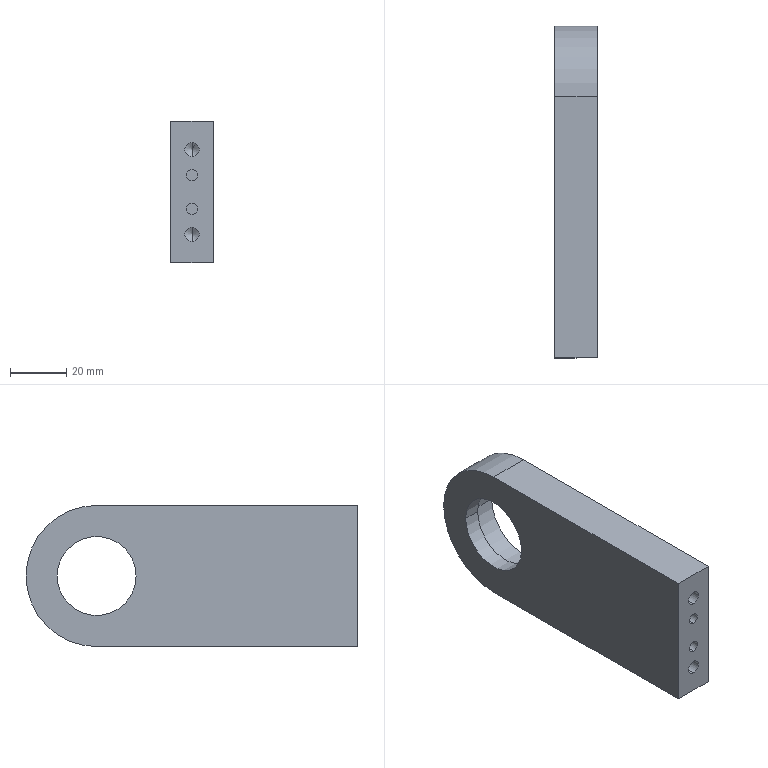Component | SolidWorks | 02-1 | 1 solid | 25 faces | box 15 x 117.6 x 50 mm | volume 72305 mm3 | cylinder 13 | plane 8 | cone 4 | commonest cylinder face diameters 4 x4 5 x4 32 x2 28 x2 50 x1
build123d program:
from build123d import *

# Parameters (mm, degrees)
SKETCH1_W             = 50
SKETCH1_H             = 117.6
EXTRUDE1_DEPTH        = 7.5
EXTRUDE3_DEPTH        = 66.631
SKETCH2_R             = 14
EXTRUDE2_DEPTH        = 66.631
SKETCH8_R             = 16
CUT_EXTRUDE1_DEPTH    = 9
M6_TAPPED_HOLE1_D     = 5
M6_TAPPED_HOLE1_DEPTH = 17
M6_TAPPED_HOLE1_TIP   = 1.502
SKETCH3_2_R           = 2
CUT_EXTRUDE1_2_DEPTH  = 10


with BuildPart() as part:
    # Sketch1 → Extrude1 (new, symmetric)
    with BuildSketch(Plane(origin=(0, 0, 0), x_dir=(1, 0, 0), z_dir=(0, 1, 0))):
        Rectangle(SKETCH1_W, SKETCH1_H)
    extrude(amount=EXTRUDE1_DEPTH, both=True)

    # Sketch3 → Extrude3 (cut, through all)
    with BuildSketch(Plane(origin=(0, 7.5, 0), x_dir=(1, 0, 0), z_dir=(0, 1, 0))):
        with BuildLine():
            ThreePointArc((0, 58.8), (17.678, 51.478), (25, 33.8))
            Line((25, 33.8), (25, 58.8))
            Line((25, 58.8), (0, 58.8))
        make_face()
        with BuildLine():
            ThreePointArc((-25, 33.8), (-17.678, 51.478), (0, 58.8))
            Line((0, 58.8), (-25, 58.8))
            Line((-25, 58.8), (-25, 33.8))
        make_face()
    extrude(amount=-EXTRUDE3_DEPTH, mode=Mode.SUBTRACT)

    # Sketch2 → Extrude2 (cut, through all)
    with BuildSketch(Plane(origin=(0, 7.5, 0), x_dir=(1, 0, 0), z_dir=(0, 1, 0))):
        with Locations(Location((0, 33.8, 0), (0, 0, 270))):
            Circle(SKETCH2_R)
    extrude(amount=-EXTRUDE2_DEPTH, mode=Mode.SUBTRACT)

    # Sketch8 → Cut-Extrude1 (cut)
    with BuildSketch(Plane.XZ.offset(7.5)):
        with Locations(Location((0, -33.8, 0), (0, 0, 270))):
            Circle(SKETCH8_R)
    extrude(amount=-CUT_EXTRUDE1_DEPTH, mode=Mode.SUBTRACT)

    # M6 Tapped Hole1
    with Locations(Plane.XY.offset(58.8)):
        with Locations((15, 0), (-15, 0)):
            Hole(M6_TAPPED_HOLE1_D / 2, depth=M6_TAPPED_HOLE1_DEPTH)
            with Locations((0, 0, -(M6_TAPPED_HOLE1_DEPTH + M6_TAPPED_HOLE1_TIP / 2))):  # 118° drill point
                Cone(0, M6_TAPPED_HOLE1_D / 2, M6_TAPPED_HOLE1_TIP, mode=Mode.SUBTRACT)

    # Sketch3_2 → Cut-Extrude1_2 (cut)
    with BuildSketch(Plane.XY.offset(58.8)):
        with Locations((6, 0)):
            Circle(SKETCH3_2_R)
        with Locations((-6, 0)):
            Circle(SKETCH3_2_R)
    extrude(amount=-CUT_EXTRUDE1_2_DEPTH, mode=Mode.SUBTRACT)


solid = part.part

# Placed as in the assembly
solid = solid.moved(Location((-87, -66.3, 30), (90, 0, 90)))
STEP:
#1=COLOUR_RGB('',0.7922,0.8196,0.9333);
#2=FILL_AREA_STYLE_COLOUR('',#1);
#3=FILL_AREA_STYLE('',(#2));
#4=SURFACE_STYLE_FILL_AREA(#3);
#5=SURFACE_SIDE_STYLE('',(#4));
#6=SURFACE_STYLE_USAGE(.BOTH.,#5);
#7=PRESENTATION_STYLE_ASSIGNMENT((#6));
#8=CARTESIAN_POINT('',(-3.425,-4.531,0.8661));
#9=VERTEX_POINT('',#8);
#10=CARTESIAN_POINT('',(-3.425,-4.531,1.024));
#11=VERTEX_POINT('',#10);
#12=CARTESIAN_POINT('',(-3.425,-4.531,0.9449));
#13=DIRECTION('',(0.,-1.,-0.));
#14=DIRECTION('',(0.,0.,1.));
#15=AXIS2_PLACEMENT_3D('',#12,#13,#14);
#16=CIRCLE('',#15,0.07874);
#17=EDGE_CURVE('',#9,#11,#16,.T.);
#18=ORIENTED_EDGE('',*,*,#17,.F.);
#19=CARTESIAN_POINT('',(-3.425,-4.925,0.8661));
#20=VERTEX_POINT('',#19);
#21=CARTESIAN_POINT('',(-3.425,-4.531,0.8661));
#22=DIRECTION('',(0.,-1.,-0.));
#23=VECTOR('',#22,39.37);
#24=LINE('',#21,#23);
#25=EDGE_CURVE('',#9,#20,#24,.T.);
#26=ORIENTED_EDGE('',*,*,#25,.T.);
#27=CARTESIAN_POINT('',(-3.425,-4.925,1.024));
#28=VERTEX_POINT('',#27);
#29=CARTESIAN_POINT('',(-3.425,-4.925,0.9449));
#30=DIRECTION('',(0.,-1.,-0.));
#31=DIRECTION('',(0.,0.,1.));
#32=AXIS2_PLACEMENT_3D('',#29,#30,#31);
#33=CIRCLE('',#32,0.07874);
#34=EDGE_CURVE('',#20,#28,#33,.T.);
#35=ORIENTED_EDGE('',*,*,#34,.T.);
#36=CARTESIAN_POINT('',(-3.425,-4.531,1.024));
#37=DIRECTION('',(0.,-1.,-0.));
#38=VECTOR('',#37,39.37);
#39=LINE('',#36,#38);
#40=EDGE_CURVE('',#11,#28,#39,.T.);
#41=ORIENTED_EDGE('',*,*,#40,.F.);
#42=EDGE_LOOP('',(#18,#26,#35,#41));
#43=FACE_OUTER_BOUND('',#42,.T.);
#44=CARTESIAN_POINT('',(-3.425,-4.531,0.9449));
#45=DIRECTION('',(0.,-1.,-0.));
#46=DIRECTION('',(0.,0.,1.));
#47=AXIS2_PLACEMENT_3D('',#44,#45,#46);
#48=CYLINDRICAL_SURFACE('',#47,0.07874);
#49=ADVANCED_FACE('',(#43),#48,.F.);
#50=CARTESIAN_POINT('',(-3.425,-4.531,1.339));
#51=VERTEX_POINT('',#50);
#52=CARTESIAN_POINT('',(-3.425,-4.531,1.496));
#53=VERTEX_POINT('',#52);
#54=CARTESIAN_POINT('',(-3.425,-4.531,1.417));
#55=DIRECTION('',(0.,-1.,-0.));
#56=DIRECTION('',(0.,0.,1.));
#57=AXIS2_PLACEMENT_3D('',#54,#55,#56);
#58=CIRCLE('',#57,0.07874);
#59=EDGE_CURVE('',#51,#53,#58,.T.);
#60=ORIENTED_EDGE('',*,*,#59,.F.);
#61=CARTESIAN_POINT('',(-3.425,-4.925,1.339));
#62=VERTEX_POINT('',#61);
#63=CARTESIAN_POINT('',(-3.425,-4.531,1.339));
#64=DIRECTION('',(0.,-1.,-0.));
#65=VECTOR('',#64,39.37);
#66=LINE('',#63,#65);
#67=EDGE_CURVE('',#51,#62,#66,.T.);
#68=ORIENTED_EDGE('',*,*,#67,.T.);
#69=CARTESIAN_POINT('',(-3.425,-4.925,1.496));
#70=VERTEX_POINT('',#69);
#71=CARTESIAN_POINT('',(-3.425,-4.925,1.417));
#72=DIRECTION('',(0.,-1.,-0.));
#73=DIRECTION('',(0.,0.,1.));
#74=AXIS2_PLACEMENT_3D('',#71,#72,#73);
#75=CIRCLE('',#74,0.07874);
#76=EDGE_CURVE('',#62,#70,#75,.T.);
#77=ORIENTED_EDGE('',*,*,#76,.T.);
#78=CARTESIAN_POINT('',(-3.425,-4.531,1.496));
#79=DIRECTION('',(0.,-1.,-0.));
#80=VECTOR('',#79,39.37);
#81=LINE('',#78,#80);
#82=EDGE_CURVE('',#53,#70,#81,.T.);
#83=ORIENTED_EDGE('',*,*,#82,.F.);
#84=EDGE_LOOP('',(#60,#68,#77,#83));
#85=FACE_OUTER_BOUND('',#84,.T.);
#86=CARTESIAN_POINT('',(-3.425,-4.531,1.417));
#87=DIRECTION('',(0.,-1.,-0.));
#88=DIRECTION('',(0.,0.,1.));
#89=AXIS2_PLACEMENT_3D('',#86,#87,#88);
#90=CYLINDRICAL_SURFACE('',#89,0.07874);
#91=ADVANCED_FACE('',(#85),#90,.F.);
#92=CARTESIAN_POINT('',(-3.425,-4.256,1.673));
#93=VERTEX_POINT('',#92);
#94=CARTESIAN_POINT('',(-3.425,-4.256,1.87));
#95=VERTEX_POINT('',#94);
#96=CARTESIAN_POINT('',(-3.425,-4.256,1.772));
#97=DIRECTION('',(0.,-1.,-0.));
#98=DIRECTION('',(0.,0.,1.));
#99=AXIS2_PLACEMENT_3D('',#96,#97,#98);
#100=CIRCLE('',#99,0.09843);
#101=EDGE_CURVE('',#93,#95,#100,.T.);
#102=ORIENTED_EDGE('',*,*,#101,.F.);
#103=CARTESIAN_POINT('',(-3.425,-4.925,1.673));
#104=VERTEX_POINT('',#103);
#105=CARTESIAN_POINT('',(-3.425,-4.925,1.673));
#106=DIRECTION('',(0.,-1.,-0.));
#107=VECTOR('',#106,39.37);
#108=LINE('',#105,#107);
#109=EDGE_CURVE('',#93,#104,#108,.T.);
#110=ORIENTED_EDGE('',*,*,#109,.T.);
#111=CARTESIAN_POINT('',(-3.425,-4.925,1.87));
#112=VERTEX_POINT('',#111);
#113=CARTESIAN_POINT('',(-3.425,-4.925,1.772));
#114=DIRECTION('',(0.,-1.,-0.));
#115=DIRECTION('',(0.,0.,1.));
#116=AXIS2_PLACEMENT_3D('',#113,#114,#115);
#117=CIRCLE('',#116,0.09843);
#118=EDGE_CURVE('',#104,#112,#117,.T.);
#119=ORIENTED_EDGE('',*,*,#118,.T.);
#120=CARTESIAN_POINT('',(-3.425,-4.925,1.87));
#121=DIRECTION('',(0.,-1.,-0.));
#122=VECTOR('',#121,39.37);
#123=LINE('',#120,#122);
#124=EDGE_CURVE('',#95,#112,#123,.T.);
#125=ORIENTED_EDGE('',*,*,#124,.F.);
#126=EDGE_LOOP('',(#102,#110,#119,#125));
#127=FACE_OUTER_BOUND('',#126,.T.);
#128=CARTESIAN_POINT('',(-3.425,-4.925,1.772));
#129=DIRECTION('',(0.,-1.,-0.));
#130=DIRECTION('',(0.,0.,1.));
#131=AXIS2_PLACEMENT_3D('',#128,#129,#130);
#132=CYLINDRICAL_SURFACE('',#131,0.09843);
#133=ADVANCED_FACE('',(#127),#132,.F.);
#134=CARTESIAN_POINT('',(-3.425,-4.197,1.772));
#135=VERTEX_POINT('',#134);
#136=CARTESIAN_POINT('',(-3.425,-4.256,1.87));
#137=DIRECTION('',(0.,-0.515,0.8572));
#138=VECTOR('',#137,39.37);
#139=LINE('',#136,#138);
#140=EDGE_CURVE('',#135,#95,#139,.T.);
#141=ORIENTED_EDGE('',*,*,#140,.F.);
#142=CARTESIAN_POINT('',(-3.425,-4.256,1.673));
#143=DIRECTION('',(-0.,-0.515,-0.8572));
#144=VECTOR('',#143,39.37);
#145=LINE('',#142,#144);
#146=EDGE_CURVE('',#135,#93,#145,.T.);
#147=ORIENTED_EDGE('',*,*,#146,.T.);
#148=ORIENTED_EDGE('',*,*,#101,.T.);
#149=EDGE_LOOP('',(#141,#147,#148));
#150=FACE_OUTER_BOUND('',#149,.T.);
#151=CARTESIAN_POINT('',(-3.425,-4.256,1.772));
#152=DIRECTION('',(0.,-1.,-0.));
#153=DIRECTION('',(0.,0.,1.));
#154=AXIS2_PLACEMENT_3D('',#151,#152,#153);
#155=CONICAL_SURFACE('',#154,0.09843,1.03);
#156=ADVANCED_FACE('',(#150),#155,.F.);
#157=CARTESIAN_POINT('',(-3.425,-4.256,0.4921));
#158=VERTEX_POINT('',#157);
#159=CARTESIAN_POINT('',(-3.425,-4.256,0.689));
#160=VERTEX_POINT('',#159);
#161=CARTESIAN_POINT('',(-3.425,-4.256,0.5906));
#162=DIRECTION('',(0.,-1.,-0.));
#163=DIRECTION('',(0.,0.,1.));
#164=AXIS2_PLACEMENT_3D('',#161,#162,#163);
#165=CIRCLE('',#164,0.09843);
#166=EDGE_CURVE('',#158,#160,#165,.T.);
#167=ORIENTED_EDGE('',*,*,#166,.F.);
#168=CARTESIAN_POINT('',(-3.425,-4.925,0.4921));
#169=VERTEX_POINT('',#168);
#170=CARTESIAN_POINT('',(-3.425,-4.925,0.4921));
#171=DIRECTION('',(0.,-1.,-0.));
#172=VECTOR('',#171,39.37);
#173=LINE('',#170,#172);
#174=EDGE_CURVE('',#158,#169,#173,.T.);
#175=ORIENTED_EDGE('',*,*,#174,.T.);
#176=CARTESIAN_POINT('',(-3.425,-4.925,0.689));
#177=VERTEX_POINT('',#176);
#178=CARTESIAN_POINT('',(-3.425,-4.925,0.5906));
#179=DIRECTION('',(0.,-1.,-0.));
#180=DIRECTION('',(0.,0.,1.));
#181=AXIS2_PLACEMENT_3D('',#178,#179,#180);
#182=CIRCLE('',#181,0.09843);
#183=EDGE_CURVE('',#169,#177,#182,.T.);
#184=ORIENTED_EDGE('',*,*,#183,.T.);
#185=CARTESIAN_POINT('',(-3.425,-4.925,0.689));
#186=DIRECTION('',(0.,-1.,-0.));
#187=VECTOR('',#186,39.37);
#188=LINE('',#185,#187);
#189=EDGE_CURVE('',#160,#177,#188,.T.);
#190=ORIENTED_EDGE('',*,*,#189,.F.);
#191=EDGE_LOOP('',(#167,#175,#184,#190));
#192=FACE_OUTER_BOUND('',#191,.T.);
#193=CARTESIAN_POINT('',(-3.425,-4.925,0.5906));
#194=DIRECTION('',(0.,-1.,-0.));
#195=DIRECTION('',(0.,0.,1.));
#196=AXIS2_PLACEMENT_3D('',#193,#194,#195);
#197=CYLINDRICAL_SURFACE('',#196,0.09843);
#198=ADVANCED_FACE('',(#192),#197,.F.);
#199=CARTESIAN_POINT('',(-3.425,-4.197,0.5906));
#200=VERTEX_POINT('',#199);
#201=CARTESIAN_POINT('',(-3.425,-4.256,0.689));
#202=DIRECTION('',(0.,-0.515,0.8572));
#203=VECTOR('',#202,39.37);
#204=LINE('',#201,#203);
#205=EDGE_CURVE('',#200,#160,#204,.T.);
#206=ORIENTED_EDGE('',*,*,#205,.F.);
#207=CARTESIAN_POINT('',(-3.425,-4.256,0.4921));
#208=DIRECTION('',(-0.,-0.515,-0.8572));
#209=VECTOR('',#208,39.37);
#210=LINE('',#207,#209);
#211=EDGE_CURVE('',#200,#158,#210,.T.);
#212=ORIENTED_EDGE('',*,*,#211,.T.);
#213=ORIENTED_EDGE('',*,*,#166,.T.);
#214=EDGE_LOOP('',(#206,#212,#213));
#215=FACE_OUTER_BOUND('',#214,.T.);
#216=CARTESIAN_POINT('',(-3.425,-4.256,0.5906));
#217=DIRECTION('',(0.,-1.,-0.));
#218=DIRECTION('',(0.,0.,1.));
#219=AXIS2_PLACEMENT_3D('',#216,#217,#218);
#220=CONICAL_SURFACE('',#219,0.09843,1.03);
#221=ADVANCED_FACE('',(#215),#220,.F.);
#222=CARTESIAN_POINT('',(-3.484,-1.909,1.181));
#223=VERTEX_POINT('',#222);
#224=CARTESIAN_POINT('',(-3.484,-0.6496,1.181));
#225=VERTEX_POINT('',#224);
#226=CARTESIAN_POINT('',(-3.484,-1.28,1.181));
#227=DIRECTION('',(1.,0.,-0.));
#228=DIRECTION('',(0.,1.,0.));
#229=AXIS2_PLACEMENT_3D('',#226,#227,#228);
#230=CIRCLE('',#229,0.6299);
#231=EDGE_CURVE('',#223,#225,#230,.T.);
#232=ORIENTED_EDGE('',*,*,#231,.F.);
#233=CARTESIAN_POINT('',(-3.13,-1.909,1.181));
#234=VERTEX_POINT('',#233);
#235=CARTESIAN_POINT('',(-3.484,-1.909,1.181));
#236=DIRECTION('',(1.,0.,-0.));
#237=VECTOR('',#236,39.37);
#238=LINE('',#235,#237);
#239=EDGE_CURVE('',#223,#234,#238,.T.);
#240=ORIENTED_EDGE('',*,*,#239,.T.);
#241=CARTESIAN_POINT('',(-3.13,-0.6496,1.181));
#242=VERTEX_POINT('',#241);
#243=CARTESIAN_POINT('',(-3.13,-1.28,1.181));
#244=DIRECTION('',(1.,0.,-0.));
#245=DIRECTION('',(0.,1.,0.));
#246=AXIS2_PLACEMENT_3D('',#243,#244,#245);
#247=CIRCLE('',#246,0.6299);
#248=EDGE_CURVE('',#234,#242,#247,.T.);
#249=ORIENTED_EDGE('',*,*,#248,.T.);
#250=CARTESIAN_POINT('',(-3.484,-0.6496,1.181));
#251=DIRECTION('',(1.,0.,-0.));
#252=VECTOR('',#251,39.37);
#253=LINE('',#250,#252);
#254=EDGE_CURVE('',#225,#242,#253,.T.);
#255=ORIENTED_EDGE('',*,*,#254,.F.);
#256=EDGE_LOOP('',(#232,#240,#249,#255));
#257=FACE_OUTER_BOUND('',#256,.T.);
#258=CARTESIAN_POINT('',(-3.484,-1.28,1.181));
#259=DIRECTION('',(1.,0.,-0.));
#260=DIRECTION('',(0.,1.,0.));
#261=AXIS2_PLACEMENT_3D('',#258,#259,#260);
#262=CYLINDRICAL_SURFACE('',#261,0.6299);
#263=ADVANCED_FACE('',(#257),#262,.F.);
#264=CARTESIAN_POINT('',(-3.484,-0.7283,1.181));
#265=VERTEX_POINT('',#264);
#266=CARTESIAN_POINT('',(-3.484,-1.831,1.181));
#267=VERTEX_POINT('',#266);
#268=CARTESIAN_POINT('',(-3.484,-1.28,1.181));
#269=DIRECTION('',(-1.,-0.,0.));
#270=DIRECTION('',(0.,1.,0.));
#271=AXIS2_PLACEMENT_3D('',#268,#269,#270);
#272=CIRCLE('',#271,0.5512);
#273=EDGE_CURVE('',#265,#267,#272,.T.);
#274=ORIENTED_EDGE('',*,*,#273,.F.);
#275=CARTESIAN_POINT('',(-3.72,-0.7283,1.181));
#276=VERTEX_POINT('',#275);
#277=CARTESIAN_POINT('',(-3.13,-0.7283,1.181));
#278=DIRECTION('',(-1.,-0.,0.));
#279=VECTOR('',#278,39.37);
#280=LINE('',#277,#279);
#281=EDGE_CURVE('',#265,#276,#280,.T.);
#282=ORIENTED_EDGE('',*,*,#281,.T.);
#283=CARTESIAN_POINT('',(-3.72,-1.831,1.181));
#284=VERTEX_POINT('',#283);
#285=CARTESIAN_POINT('',(-3.72,-1.28,1.181));
#286=DIRECTION('',(-1.,-0.,0.));
#287=DIRECTION('',(0.,-1.,0.));
#288=AXIS2_PLACEMENT_3D('',#285,#286,#287);
#289=CIRCLE('',#288,0.5512);
#290=EDGE_CURVE('',#276,#284,#289,.T.);
#291=ORIENTED_EDGE('',*,*,#290,.T.);
#292=CARTESIAN_POINT('',(-3.13,-1.831,1.181));
#293=DIRECTION('',(-1.,-0.,0.));
#294=VECTOR('',#293,39.37);
#295=LINE('',#292,#294);
#296=EDGE_CURVE('',#267,#284,#295,.T.);
#297=ORIENTED_EDGE('',*,*,#296,.F.);
#298=EDGE_LOOP('',(#274,#282,#291,#297));
#299=FACE_OUTER_BOUND('',#298,.T.);
#300=CARTESIAN_POINT('',(-3.13,-1.28,1.181));
#301=DIRECTION('',(-1.,-0.,0.));
#302=DIRECTION('',(0.,-1.,0.));
#303=AXIS2_PLACEMENT_3D('',#300,#301,#302);
#304=CYLINDRICAL_SURFACE('',#303,0.5512);
#305=ADVANCED_FACE('',(#299),#304,.F.);
#306=ORIENTED_EDGE('',*,*,#281,.F.);
#307=CARTESIAN_POINT('',(-3.484,-1.28,1.181));
#308=DIRECTION('',(-1.,-0.,0.));
#309=DIRECTION('',(0.,1.,0.));
#310=AXIS2_PLACEMENT_3D('',#307,#308,#309);
#311=CIRCLE('',#310,0.5512);
#312=EDGE_CURVE('',#267,#265,#311,.T.);
#313=ORIENTED_EDGE('',*,*,#312,.F.);
#314=ORIENTED_EDGE('',*,*,#296,.T.);
#315=CARTESIAN_POINT('',(-3.72,-1.28,1.181));
#316=DIRECTION('',(-1.,-0.,0.));
#317=DIRECTION('',(0.,-1.,0.));
#318=AXIS2_PLACEMENT_3D('',#315,#316,#317);
#319=CIRCLE('',#318,0.5512);
#320=EDGE_CURVE('',#284,#276,#319,.T.);
#321=ORIENTED_EDGE('',*,*,#320,.T.);
#322=EDGE_LOOP('',(#306,#313,#314,#321));
#323=FACE_OUTER_BOUND('',#322,.T.);
#324=CARTESIAN_POINT('',(-3.13,-1.28,1.181));
#325=DIRECTION('',(-1.,-0.,0.));
#326=DIRECTION('',(0.,-1.,0.));
#327=AXIS2_PLACEMENT_3D('',#324,#325,#326);
#328=CYLINDRICAL_SURFACE('',#327,0.5512);
#329=ADVANCED_FACE('',(#323),#328,.F.);
#330=ORIENTED_EDGE('',*,*,#320,.F.);
#331=ORIENTED_EDGE('',*,*,#290,.F.);
#332=EDGE_LOOP('',(#330,#331));
#333=FACE_BOUND('',#332,.T.);
#334=CARTESIAN_POINT('',(-3.72,-4.925,2.165));
#335=VERTEX_POINT('',#334);
#336=CARTESIAN_POINT('',(-3.72,-1.28,2.165));
#337=VERTEX_POINT('',#336);
#338=CARTESIAN_POINT('',(-3.72,-0.2953,2.165));
#339=DIRECTION('',(-0.,1.,0.));
#340=VECTOR('',#339,39.37);
#341=LINE('',#338,#340);
#342=EDGE_CURVE('',#335,#337,#341,.T.);
#343=ORIENTED_EDGE('',*,*,#342,.T.);
#344=CARTESIAN_POINT('',(-3.72,-1.28,0.1969));
#345=VERTEX_POINT('',#344);
#346=CARTESIAN_POINT('',(-3.72,-1.28,1.181));
#347=DIRECTION('',(-1.,-0.,0.));
#348=DIRECTION('',(0.,-1.,-0.));
#349=AXIS2_PLACEMENT_3D('',#346,#347,#348);
#350=CIRCLE('',#349,0.9843);
#351=EDGE_CURVE('',#337,#345,#350,.T.);
#352=ORIENTED_EDGE('',*,*,#351,.T.);
#353=CARTESIAN_POINT('',(-3.72,-4.925,0.1969));
#354=VERTEX_POINT('',#353);
#355=CARTESIAN_POINT('',(-3.72,-0.2953,0.1969));
#356=DIRECTION('',(0.,-1.,-0.));
#357=VECTOR('',#356,39.37);
#358=LINE('',#355,#357);
#359=EDGE_CURVE('',#345,#354,#358,.T.);
#360=ORIENTED_EDGE('',*,*,#359,.T.);
#361=CARTESIAN_POINT('',(-3.72,-4.925,2.165));
#362=DIRECTION('',(0.,-0.,1.));
#363=VECTOR('',#362,39.37);
#364=LINE('',#361,#363);
#365=EDGE_CURVE('',#354,#335,#364,.T.);
#366=ORIENTED_EDGE('',*,*,#365,.T.);
#367=EDGE_LOOP('',(#343,#352,#360,#366));
#368=FACE_OUTER_BOUND('',#367,.T.);
#369=CARTESIAN_POINT('',(-3.72,-2.61,1.181));
#370=DIRECTION('',(1.,0.,-0.));
#371=DIRECTION('',(-0.,1.,0.));
#372=AXIS2_PLACEMENT_3D('',#369,#370,#371);
#373=PLANE('',#372);
#374=ADVANCED_FACE('',(#333,#368),#373,.F.);
#375=CARTESIAN_POINT('',(-3.13,-1.28,1.181));
#376=DIRECTION('',(1.,0.,-0.));
#377=DIRECTION('',(0.,1.,0.));
#378=AXIS2_PLACEMENT_3D('',#375,#376,#377);
#379=CIRCLE('',#378,0.6299);
#380=EDGE_CURVE('',#242,#234,#379,.T.);
#381=ORIENTED_EDGE('',*,*,#380,.F.);
#382=ORIENTED_EDGE('',*,*,#248,.F.);
#383=EDGE_LOOP('',(#381,#382));
#384=FACE_BOUND('',#383,.T.);
#385=CARTESIAN_POINT('',(-3.13,-1.28,2.165));
#386=VERTEX_POINT('',#385);
#387=CARTESIAN_POINT('',(-3.13,-1.28,0.1969));
#388=VERTEX_POINT('',#387);
#389=CARTESIAN_POINT('',(-3.13,-1.28,1.181));
#390=DIRECTION('',(-1.,-0.,0.));
#391=DIRECTION('',(0.,-1.,-0.));
#392=AXIS2_PLACEMENT_3D('',#389,#390,#391);
#393=CIRCLE('',#392,0.9843);
#394=EDGE_CURVE('',#386,#388,#393,.T.);
#395=ORIENTED_EDGE('',*,*,#394,.F.);
#396=CARTESIAN_POINT('',(-3.13,-4.925,2.165));
#397=VERTEX_POINT('',#396);
#398=CARTESIAN_POINT('',(-3.13,-0.2953,2.165));
#399=DIRECTION('',(-0.,1.,0.));
#400=VECTOR('',#399,39.37);
#401=LINE('',#398,#400);
#402=EDGE_CURVE('',#397,#386,#401,.T.);
#403=ORIENTED_EDGE('',*,*,#402,.F.);
#404=CARTESIAN_POINT('',(-3.13,-4.925,0.1969));
#405=VERTEX_POINT('',#404);
#406=CARTESIAN_POINT('',(-3.13,-4.925,2.165));
#407=DIRECTION('',(0.,-0.,1.));
#408=VECTOR('',#407,39.37);
#409=LINE('',#406,#408);
#410=EDGE_CURVE('',#405,#397,#409,.T.);
#411=ORIENTED_EDGE('',*,*,#410,.F.);
#412=CARTESIAN_POINT('',(-3.13,-0.2953,0.1969));
#413=DIRECTION('',(0.,-1.,-0.));
#414=VECTOR('',#413,39.37);
#415=LINE('',#412,#414);
#416=EDGE_CURVE('',#388,#405,#415,.T.);
#417=ORIENTED_EDGE('',*,*,#416,.F.);
#418=EDGE_LOOP('',(#395,#403,#411,#417));
#419=FACE_OUTER_BOUND('',#418,.T.);
#420=CARTESIAN_POINT('',(-3.13,-2.61,1.181));
#421=DIRECTION('',(1.,0.,-0.));
#422=DIRECTION('',(-0.,1.,0.));
#423=AXIS2_PLACEMENT_3D('',#420,#421,#422);
#424=PLANE('',#423);
#425=ADVANCED_FACE('',(#384,#419),#424,.T.);
#426=CARTESIAN_POINT('',(-3.13,-1.28,0.1969));
#427=DIRECTION('',(-1.,-0.,0.));
#428=VECTOR('',#427,39.37);
#429=LINE('',#426,#428);
#430=EDGE_CURVE('',#388,#345,#429,.T.);
#431=ORIENTED_EDGE('',*,*,#430,.F.);
#432=ORIENTED_EDGE('',*,*,#416,.T.);
#433=CARTESIAN_POINT('',(-3.72,-4.925,0.1969));
#434=DIRECTION('',(1.,0.,-0.));
#435=VECTOR('',#434,39.37);
#436=LINE('',#433,#435);
#437=EDGE_CURVE('',#354,#405,#436,.T.);
#438=ORIENTED_EDGE('',*,*,#437,.F.);
#439=ORIENTED_EDGE('',*,*,#359,.F.);
#440=EDGE_LOOP('',(#431,#432,#438,#439));
#441=FACE_OUTER_BOUND('',#440,.T.);
#442=CARTESIAN_POINT('',(-3.72,-0.2953,0.1969));
#443=DIRECTION('',(0.,-0.,1.));
#444=DIRECTION('',(-0.,1.,0.));
#445=AXIS2_PLACEMENT_3D('',#442,#443,#444);
#446=PLANE('',#445);
#447=ADVANCED_FACE('',(#441),#446,.F.);
#448=ORIENTED_EDGE('',*,*,#402,.T.);
#449=CARTESIAN_POINT('',(-3.13,-1.28,2.165));
#450=DIRECTION('',(-1.,-0.,0.));
#451=VECTOR('',#450,39.37);
#452=LINE('',#449,#451);
#453=EDGE_CURVE('',#386,#337,#452,.T.);
#454=ORIENTED_EDGE('',*,*,#453,.T.);
#455=ORIENTED_EDGE('',*,*,#342,.F.);
#456=CARTESIAN_POINT('',(-3.72,-4.925,2.165));
#457=DIRECTION('',(1.,0.,-0.));
#458=VECTOR('',#457,39.37);
#459=LINE('',#456,#458);
#460=EDGE_CURVE('',#335,#397,#459,.T.);
#461=ORIENTED_EDGE('',*,*,#460,.T.);
#462=EDGE_LOOP('',(#448,#454,#455,#461));
#463=FACE_OUTER_BOUND('',#462,.T.);
#464=CARTESIAN_POINT('',(-3.72,-0.2953,2.165));
#465=DIRECTION('',(-0.,0.,-1.));
#466=DIRECTION('',(0.,-1.,-0.));
#467=AXIS2_PLACEMENT_3D('',#464,#465,#466);
#468=PLANE('',#467);
#469=ADVANCED_FACE('',(#463),#468,.F.);
#470=CARTESIAN_POINT('',(-3.425,-4.925,0.9449));
#471=DIRECTION('',(0.,-1.,-0.));
#472=DIRECTION('',(0.,0.,1.));
#473=AXIS2_PLACEMENT_3D('',#470,#471,#472);
#474=CIRCLE('',#473,0.07874);
#475=EDGE_CURVE('',#28,#20,#474,.T.);
#476=ORIENTED_EDGE('',*,*,#475,.F.);
#477=ORIENTED_EDGE('',*,*,#34,.F.);
#478=EDGE_LOOP('',(#476,#477));
#479=FACE_BOUND('',#478,.T.);
#480=CARTESIAN_POINT('',(-3.425,-4.925,1.417));
#481=DIRECTION('',(0.,-1.,-0.));
#482=DIRECTION('',(0.,0.,1.));
#483=AXIS2_PLACEMENT_3D('',#480,#481,#482);
#484=CIRCLE('',#483,0.07874);
#485=EDGE_CURVE('',#70,#62,#484,.T.);
#486=ORIENTED_EDGE('',*,*,#485,.F.);
#487=ORIENTED_EDGE('',*,*,#76,.F.);
#488=EDGE_LOOP('',(#486,#487));
#489=FACE_BOUND('',#488,.T.);
#490=CARTESIAN_POINT('',(-3.425,-4.925,1.772));
#491=DIRECTION('',(0.,-1.,-0.));
#492=DIRECTION('',(0.,0.,1.));
#493=AXIS2_PLACEMENT_3D('',#490,#491,#492);
#494=CIRCLE('',#493,0.09843);
#495=EDGE_CURVE('',#112,#104,#494,.T.);
#496=ORIENTED_EDGE('',*,*,#495,.F.);
#497=ORIENTED_EDGE('',*,*,#118,.F.);
#498=EDGE_LOOP('',(#496,#497));
#499=FACE_BOUND('',#498,.T.);
#500=CARTESIAN_POINT('',(-3.425,-4.925,0.5906));
#501=DIRECTION('',(0.,-1.,-0.));
#502=DIRECTION('',(0.,0.,1.));
#503=AXIS2_PLACEMENT_3D('',#500,#501,#502);
#504=CIRCLE('',#503,0.09843);
#505=EDGE_CURVE('',#177,#169,#504,.T.);
#506=ORIENTED_EDGE('',*,*,#505,.F.);
#507=ORIENTED_EDGE('',*,*,#183,.F.);
#508=EDGE_LOOP('',(#506,#507));
#509=FACE_BOUND('',#508,.T.);
#510=ORIENTED_EDGE('',*,*,#410,.T.);
#511=ORIENTED_EDGE('',*,*,#460,.F.);
#512=ORIENTED_EDGE('',*,*,#365,.F.);
#513=ORIENTED_EDGE('',*,*,#437,.T.);
#514=EDGE_LOOP('',(#510,#511,#512,#513));
#515=FACE_OUTER_BOUND('',#514,.T.);
#516=CARTESIAN_POINT('',(-3.72,-4.925,2.165));
#517=DIRECTION('',(-0.,1.,0.));
#518=DIRECTION('',(-0.,0.,-1.));
#519=AXIS2_PLACEMENT_3D('',#516,#517,#518);
#520=PLANE('',#519);
#521=ADVANCED_FACE('',(#479,#489,#499,#509,#515),#520,.F.);
#522=ORIENTED_EDGE('',*,*,#351,.F.);
#523=ORIENTED_EDGE('',*,*,#453,.F.);
#524=ORIENTED_EDGE('',*,*,#394,.T.);
#525=ORIENTED_EDGE('',*,*,#430,.T.);
#526=EDGE_LOOP('',(#522,#523,#524,#525));
#527=FACE_OUTER_BOUND('',#526,.T.);
#528=CARTESIAN_POINT('',(-3.13,-1.28,1.181));
#529=DIRECTION('',(-1.,-0.,0.));
#530=DIRECTION('',(0.,-1.,-0.));
#531=AXIS2_PLACEMENT_3D('',#528,#529,#530);
#532=CYLINDRICAL_SURFACE('',#531,0.9843);
#533=ADVANCED_FACE('',(#527),#532,.T.);
#534=CARTESIAN_POINT('',(-3.484,-1.28,1.181));
#535=DIRECTION('',(1.,0.,-0.));
#536=DIRECTION('',(0.,1.,0.));
#537=AXIS2_PLACEMENT_3D('',#534,#535,#536);
#538=CIRCLE('',#537,0.6299);
#539=EDGE_CURVE('',#225,#223,#538,.T.);
#540=ORIENTED_EDGE('',*,*,#539,.T.);
#541=ORIENTED_EDGE('',*,*,#231,.T.);
#542=EDGE_LOOP('',(#540,#541));
#543=FACE_OUTER_BOUND('',#542,.T.);
#544=ORIENTED_EDGE('',*,*,#312,.T.);
#545=ORIENTED_EDGE('',*,*,#273,.T.);
#546=EDGE_LOOP('',(#544,#545));
#547=FACE_BOUND('',#546,.T.);
#548=CARTESIAN_POINT('',(-3.484,-1.28,1.181));
#549=DIRECTION('',(1.,0.,-0.));
#550=DIRECTION('',(-0.,1.,0.));
#551=AXIS2_PLACEMENT_3D('',#548,#549,#550);
#552=PLANE('',#551);
#553=ADVANCED_FACE('',(#543,#547),#552,.T.);
#554=ORIENTED_EDGE('',*,*,#239,.F.);
#555=ORIENTED_EDGE('',*,*,#539,.F.);
#556=ORIENTED_EDGE('',*,*,#254,.T.);
#557=ORIENTED_EDGE('',*,*,#380,.T.);
#558=EDGE_LOOP('',(#554,#555,#556,#557));
#559=FACE_OUTER_BOUND('',#558,.T.);
#560=CARTESIAN_POINT('',(-3.484,-1.28,1.181));
#561=DIRECTION('',(1.,0.,-0.));
#562=DIRECTION('',(0.,1.,0.));
#563=AXIS2_PLACEMENT_3D('',#560,#561,#562);
#564=CYLINDRICAL_SURFACE('',#563,0.6299);
#565=ADVANCED_FACE('',(#559),#564,.F.);
#566=ORIENTED_EDGE('',*,*,#211,.F.);
#567=ORIENTED_EDGE('',*,*,#205,.T.);
#568=CARTESIAN_POINT('',(-3.425,-4.256,0.5906));
#569=DIRECTION('',(0.,-1.,-0.));
#570=DIRECTION('',(0.,0.,1.));
#571=AXIS2_PLACEMENT_3D('',#568,#569,#570);
#572=CIRCLE('',#571,0.09843);
#573=EDGE_CURVE('',#160,#158,#572,.T.);
#574=ORIENTED_EDGE('',*,*,#573,.T.);
#575=EDGE_LOOP('',(#566,#567,#574));
#576=FACE_OUTER_BOUND('',#575,.T.);
#577=CARTESIAN_POINT('',(-3.425,-4.256,0.5906));
#578=DIRECTION('',(0.,-1.,-0.));
#579=DIRECTION('',(0.,0.,1.));
#580=AXIS2_PLACEMENT_3D('',#577,#578,#579);
#581=CONICAL_SURFACE('',#580,0.09843,1.03);
#582=ADVANCED_FACE('',(#576),#581,.F.);
#583=ORIENTED_EDGE('',*,*,#174,.F.);
#584=ORIENTED_EDGE('',*,*,#573,.F.);
#585=ORIENTED_EDGE('',*,*,#189,.T.);
#586=ORIENTED_EDGE('',*,*,#505,.T.);
#587=EDGE_LOOP('',(#583,#584,#585,#586));
#588=FACE_OUTER_BOUND('',#587,.T.);
#589=CARTESIAN_POINT('',(-3.425,-4.925,0.5906));
#590=DIRECTION('',(0.,-1.,-0.));
#591=DIRECTION('',(0.,0.,1.));
#592=AXIS2_PLACEMENT_3D('',#589,#590,#591);
#593=CYLINDRICAL_SURFACE('',#592,0.09843);
#594=ADVANCED_FACE('',(#588),#593,.F.);
#595=ORIENTED_EDGE('',*,*,#146,.F.);
#596=ORIENTED_EDGE('',*,*,#140,.T.);
#597=CARTESIAN_POINT('',(-3.425,-4.256,1.772));
#598=DIRECTION('',(0.,-1.,-0.));
#599=DIRECTION('',(0.,0.,1.));
#600=AXIS2_PLACEMENT_3D('',#597,#598,#599);
#601=CIRCLE('',#600,0.09843);
#602=EDGE_CURVE('',#95,#93,#601,.T.);
#603=ORIENTED_EDGE('',*,*,#602,.T.);
#604=EDGE_LOOP('',(#595,#596,#603));
#605=FACE_OUTER_BOUND('',#604,.T.);
#606=CARTESIAN_POINT('',(-3.425,-4.256,1.772));
#607=DIRECTION('',(0.,-1.,-0.));
#608=DIRECTION('',(0.,0.,1.));
#609=AXIS2_PLACEMENT_3D('',#606,#607,#608);
#610=CONICAL_SURFACE('',#609,0.09843,1.03);
#611=ADVANCED_FACE('',(#605),#610,.F.);
#612=ORIENTED_EDGE('',*,*,#109,.F.);
#613=ORIENTED_EDGE('',*,*,#602,.F.);
#614=ORIENTED_EDGE('',*,*,#124,.T.);
#615=ORIENTED_EDGE('',*,*,#495,.T.);
#616=EDGE_LOOP('',(#612,#613,#614,#615));
#617=FACE_OUTER_BOUND('',#616,.T.);
#618=CARTESIAN_POINT('',(-3.425,-4.925,1.772));
#619=DIRECTION('',(0.,-1.,-0.));
#620=DIRECTION('',(0.,0.,1.));
#621=AXIS2_PLACEMENT_3D('',#618,#619,#620);
#622=CYLINDRICAL_SURFACE('',#621,0.09843);
#623=ADVANCED_FACE('',(#617),#622,.F.);
#624=ORIENTED_EDGE('',*,*,#67,.F.);
#625=CARTESIAN_POINT('',(-3.425,-4.531,1.417));
#626=DIRECTION('',(0.,-1.,-0.));
#627=DIRECTION('',(0.,0.,1.));
#628=AXIS2_PLACEMENT_3D('',#625,#626,#627);
#629=CIRCLE('',#628,0.07874);
#630=EDGE_CURVE('',#53,#51,#629,.T.);
#631=ORIENTED_EDGE('',*,*,#630,.F.);
#632=ORIENTED_EDGE('',*,*,#82,.T.);
#633=ORIENTED_EDGE('',*,*,#485,.T.);
#634=EDGE_LOOP('',(#624,#631,#632,#633));
#635=FACE_OUTER_BOUND('',#634,.T.);
#636=CARTESIAN_POINT('',(-3.425,-4.531,1.417));
#637=DIRECTION('',(0.,-1.,-0.));
#638=DIRECTION('',(0.,0.,1.));
#639=AXIS2_PLACEMENT_3D('',#636,#637,#638);
#640=CYLINDRICAL_SURFACE('',#639,0.07874);
#641=ADVANCED_FACE('',(#635),#640,.F.);
#642=ORIENTED_EDGE('',*,*,#630,.T.);
#643=ORIENTED_EDGE('',*,*,#59,.T.);
#644=EDGE_LOOP('',(#642,#643));
#645=FACE_OUTER_BOUND('',#644,.T.);
#646=CARTESIAN_POINT('',(-3.425,-4.531,1.417));
#647=DIRECTION('',(0.,-1.,-0.));
#648=DIRECTION('',(0.,-0.,1.));
#649=AXIS2_PLACEMENT_3D('',#646,#647,#648);
#650=PLANE('',#649);
#651=ADVANCED_FACE('',(#645),#650,.T.);
#652=ORIENTED_EDGE('',*,*,#25,.F.);
#653=CARTESIAN_POINT('',(-3.425,-4.531,0.9449));
#654=DIRECTION('',(0.,-1.,-0.));
#655=DIRECTION('',(0.,0.,1.));
#656=AXIS2_PLACEMENT_3D('',#653,#654,#655);
#657=CIRCLE('',#656,0.07874);
#658=EDGE_CURVE('',#11,#9,#657,.T.);
#659=ORIENTED_EDGE('',*,*,#658,.F.);
#660=ORIENTED_EDGE('',*,*,#40,.T.);
#661=ORIENTED_EDGE('',*,*,#475,.T.);
#662=EDGE_LOOP('',(#652,#659,#660,#661));
#663=FACE_OUTER_BOUND('',#662,.T.);
#664=CARTESIAN_POINT('',(-3.425,-4.531,0.9449));
#665=DIRECTION('',(0.,-1.,-0.));
#666=DIRECTION('',(0.,0.,1.));
#667=AXIS2_PLACEMENT_3D('',#664,#665,#666);
#668=CYLINDRICAL_SURFACE('',#667,0.07874);
#669=ADVANCED_FACE('',(#663),#668,.F.);
#670=ORIENTED_EDGE('',*,*,#658,.T.);
#671=ORIENTED_EDGE('',*,*,#17,.T.);
#672=EDGE_LOOP('',(#670,#671));
#673=FACE_OUTER_BOUND('',#672,.T.);
#674=CARTESIAN_POINT('',(-3.425,-4.531,0.9449));
#675=DIRECTION('',(0.,-1.,-0.));
#676=DIRECTION('',(0.,-0.,1.));
#677=AXIS2_PLACEMENT_3D('',#674,#675,#676);
#678=PLANE('',#677);
#679=ADVANCED_FACE('',(#673),#678,.T.);
#680=CLOSED_SHELL('',(#49,#91,#133,#156,#198,#221,#263,#305,#329,#374,#425,#447,#469,#521,#533,#553,#565,#582,#594,#611,#623,#641,#651,#669,#679));
#681=MANIFOLD_SOLID_BREP('',#680);
#682=STYLED_ITEM('',(#7),#681);
#683=(LENGTH_UNIT()NAMED_UNIT(*)SI_UNIT($,.METRE.));
#684=LENGTH_MEASURE_WITH_UNIT(LENGTH_MEASURE(0.0254),#683);
#685=DIMENSIONAL_EXPONENTS(1.,0.,0.,0.,0.,0.,0.);
#686=(CONVERSION_BASED_UNIT('',#684)LENGTH_UNIT()NAMED_UNIT(#685));
#687=UNCERTAINTY_MEASURE_WITH_UNIT(LENGTH_MEASURE(0.00001),#686,'','');
#688=(NAMED_UNIT(*)PLANE_ANGLE_UNIT()SI_UNIT($,.RADIAN.));
#689=(NAMED_UNIT(*)SI_UNIT($,.STERADIAN.)SOLID_ANGLE_UNIT());
#690=(GEOMETRIC_REPRESENTATION_CONTEXT(3)GLOBAL_UNCERTAINTY_ASSIGNED_CONTEXT((#687))GLOBAL_UNIT_ASSIGNED_CONTEXT((#686,#688,#689))REPRESENTATION_CONTEXT('',''));
#691=MECHANICAL_DESIGN_GEOMETRIC_PRESENTATION_REPRESENTATION('',(#682),#690);
#692=CARTESIAN_POINT('',(0.,0.,0.));
#693=DIRECTION('',(0.,0.,1.));
#694=DIRECTION('',(1.,0.,0.));
#695=AXIS2_PLACEMENT_3D('',#692,#693,#694);
#696=(LENGTH_UNIT()NAMED_UNIT(*)SI_UNIT($,.METRE.));
#697=LENGTH_MEASURE_WITH_UNIT(LENGTH_MEASURE(0.0254),#696);
#698=DIMENSIONAL_EXPONENTS(1.,0.,0.,0.,0.,0.,0.);
#699=(CONVERSION_BASED_UNIT('',#697)LENGTH_UNIT()NAMED_UNIT(#698));
#700=UNCERTAINTY_MEASURE_WITH_UNIT(LENGTH_MEASURE(0.00001),#699,'','');
#701=(NAMED_UNIT(*)PLANE_ANGLE_UNIT()SI_UNIT($,.RADIAN.));
#702=(NAMED_UNIT(*)SI_UNIT($,.STERADIAN.)SOLID_ANGLE_UNIT());
#703=(GEOMETRIC_REPRESENTATION_CONTEXT(3)GLOBAL_UNCERTAINTY_ASSIGNED_CONTEXT((#700))GLOBAL_UNIT_ASSIGNED_CONTEXT((#699,#701,#702))REPRESENTATION_CONTEXT('',''));
#704=ADVANCED_BREP_SHAPE_REPRESENTATION('',(#681,#695),#703);
#705=PRESENTATION_LAYER_ASSIGNMENT('','',(#682));